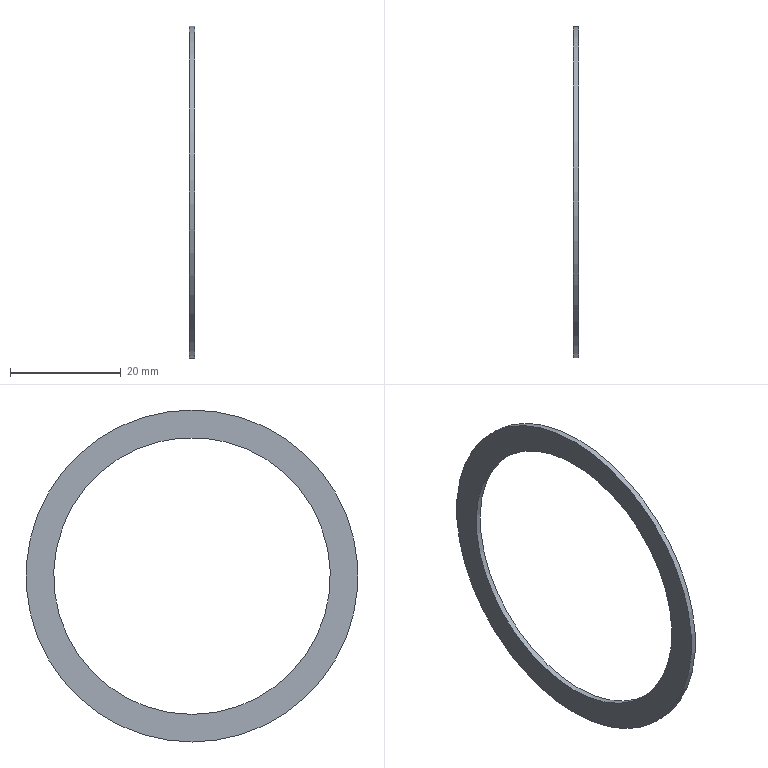Component | NX | GASKET | 1 solid | 4 faces | box 1 x 60 x 60 mm | volume 864 mm3 | cylinder 2 | plane 2 | commonest cylinder face diameters 60 x1 50 x1
STEP:
#1=CARTESIAN_POINT('',(0.,0.,0.));
#2=DIRECTION('',(0.,0.,1.));
#3=DIRECTION('',(1.,0.,0.));
#4=AXIS2_PLACEMENT_3D('',#1,#2,#3);
#5=CARTESIAN_POINT('',(144.,0.,-30.));
#6=VERTEX_POINT('',#5);
#7=CARTESIAN_POINT('',(144.,0.,0.));
#8=DIRECTION('',(1.,0.,0.));
#9=DIRECTION('',(0.,0.,-1.));
#10=AXIS2_PLACEMENT_3D('',#7,#8,#9);
#11=CIRCLE('',#10,30.);
#12=CARTESIAN_POINT('',(144.,0.,0.));
#13=DIRECTION('',(-1.,0.,0.));
#14=DIRECTION('',(0.,0.,1.));
#15=AXIS2_PLACEMENT_3D('',#12,#13,#14);
#16=CYLINDRICAL_SURFACE('',#15,30.);
#17=CARTESIAN_POINT('',(9.425,0.));
#18=DIRECTION('',(-1.,0.));
#19=VECTOR('',#18,1.);
#20=LINE('',#17,#19);
#21=(GEOMETRIC_REPRESENTATION_CONTEXT(2)PARAMETRIC_REPRESENTATION_CONTEXT()REPRESENTATION_CONTEXT('',''));
#22=DEFINITIONAL_REPRESENTATION('',(#20),#21);
#23=PCURVE('',#16,#22);
#24=CARTESIAN_POINT('',(144.,0.,0.));
#25=DIRECTION('',(1.,0.,0.));
#26=DIRECTION('',(0.,0.,-1.));
#27=AXIS2_PLACEMENT_3D('',#24,#25,#26);
#28=PLANE('',#27);
#29=CARTESIAN_POINT('',(0.,0.));
#30=DIRECTION('',(1.,0.));
#31=AXIS2_PLACEMENT_2D('',#29,#30);
#32=CIRCLE('',#31,30.);
#33=(GEOMETRIC_REPRESENTATION_CONTEXT(2)PARAMETRIC_REPRESENTATION_CONTEXT()REPRESENTATION_CONTEXT('',''));
#34=DEFINITIONAL_REPRESENTATION('',(#32),#33);
#35=PCURVE('',#28,#34);
#36=SURFACE_CURVE('',#11,(#23,#35),.PCURVE_S1.);
#37=EDGE_CURVE('',#6,#6,#36,.T.);
#38=ORIENTED_EDGE('',*,*,#37,.F.);
#39=CARTESIAN_POINT('',(143.,0.,-30.));
#40=VERTEX_POINT('',#39);
#41=CARTESIAN_POINT('',(144.,0.,-30.));
#42=CARTESIAN_POINT('',(143.,0.,-30.));
#43=B_SPLINE_CURVE_WITH_KNOTS('',1,(#41,#42),.UNSPECIFIED.,.F.,.F.,(2,2),(0.,1.),.PIECEWISE_BEZIER_KNOTS.);
#44=CARTESIAN_POINT('',(9.425,0.));
#45=DIRECTION('',(0.,1.));
#46=VECTOR('',#45,1.);
#47=LINE('',#44,#46);
#48=(GEOMETRIC_REPRESENTATION_CONTEXT(2)PARAMETRIC_REPRESENTATION_CONTEXT()REPRESENTATION_CONTEXT('',''));
#49=DEFINITIONAL_REPRESENTATION('',(#47),#48);
#50=PCURVE('',#16,#49);
#51=CARTESIAN_POINT('',(3.142,0.));
#52=DIRECTION('',(0.,1.));
#53=VECTOR('',#52,1.);
#54=LINE('',#51,#53);
#55=(GEOMETRIC_REPRESENTATION_CONTEXT(2)PARAMETRIC_REPRESENTATION_CONTEXT()REPRESENTATION_CONTEXT('',''));
#56=DEFINITIONAL_REPRESENTATION('',(#54),#55);
#57=PCURVE('',#16,#56);
#58=SEAM_CURVE('',#43,(#50,#57),.PCURVE_S1.);
#59=EDGE_CURVE('',#6,#40,#58,.T.);
#60=ORIENTED_EDGE('',*,*,#59,.T.);
#61=CARTESIAN_POINT('',(143.,0.,0.));
#62=DIRECTION('',(1.,0.,0.));
#63=DIRECTION('',(0.,0.,-1.));
#64=AXIS2_PLACEMENT_3D('',#61,#62,#63);
#65=CIRCLE('',#64,30.);
#66=CARTESIAN_POINT('',(9.425,1.));
#67=DIRECTION('',(-1.,0.));
#68=VECTOR('',#67,1.);
#69=LINE('',#66,#68);
#70=(GEOMETRIC_REPRESENTATION_CONTEXT(2)PARAMETRIC_REPRESENTATION_CONTEXT()REPRESENTATION_CONTEXT('',''));
#71=DEFINITIONAL_REPRESENTATION('',(#69),#70);
#72=PCURVE('',#16,#71);
#73=CARTESIAN_POINT('',(143.,0.,0.));
#74=DIRECTION('',(1.,0.,0.));
#75=DIRECTION('',(0.,0.,-1.));
#76=AXIS2_PLACEMENT_3D('',#73,#74,#75);
#77=PLANE('',#76);
#78=CARTESIAN_POINT('',(0.,0.));
#79=DIRECTION('',(1.,0.));
#80=AXIS2_PLACEMENT_2D('',#78,#79);
#81=CIRCLE('',#80,30.);
#82=(GEOMETRIC_REPRESENTATION_CONTEXT(2)PARAMETRIC_REPRESENTATION_CONTEXT()REPRESENTATION_CONTEXT('',''));
#83=DEFINITIONAL_REPRESENTATION('',(#81),#82);
#84=PCURVE('',#77,#83);
#85=SURFACE_CURVE('',#65,(#72,#84),.PCURVE_S1.);
#86=EDGE_CURVE('',#40,#40,#85,.T.);
#87=ORIENTED_EDGE('',*,*,#86,.T.);
#88=ORIENTED_EDGE('',*,*,#59,.F.);
#89=EDGE_LOOP('',(#38,#60,#87,#88));
#90=FACE_BOUND('',#89,.T.);
#91=ADVANCED_FACE('',(#90),#16,.T.);
#92=CARTESIAN_POINT('',(144.,0.,-25.));
#93=VERTEX_POINT('',#92);
#94=CARTESIAN_POINT('',(144.,0.,0.));
#95=DIRECTION('',(1.,0.,0.));
#96=DIRECTION('',(0.,0.,-1.));
#97=AXIS2_PLACEMENT_3D('',#94,#95,#96);
#98=CIRCLE('',#97,25.);
#99=CARTESIAN_POINT('',(144.,0.,0.));
#100=DIRECTION('',(-1.,0.,0.));
#101=DIRECTION('',(0.,0.,1.));
#102=AXIS2_PLACEMENT_3D('',#99,#100,#101);
#103=CYLINDRICAL_SURFACE('',#102,25.);
#104=CARTESIAN_POINT('',(9.425,0.));
#105=DIRECTION('',(-1.,0.));
#106=VECTOR('',#105,1.);
#107=LINE('',#104,#106);
#108=(GEOMETRIC_REPRESENTATION_CONTEXT(2)PARAMETRIC_REPRESENTATION_CONTEXT()REPRESENTATION_CONTEXT('',''));
#109=DEFINITIONAL_REPRESENTATION('',(#107),#108);
#110=PCURVE('',#103,#109);
#111=CARTESIAN_POINT('',(0.,0.));
#112=DIRECTION('',(1.,0.));
#113=AXIS2_PLACEMENT_2D('',#111,#112);
#114=CIRCLE('',#113,25.);
#115=(GEOMETRIC_REPRESENTATION_CONTEXT(2)PARAMETRIC_REPRESENTATION_CONTEXT()REPRESENTATION_CONTEXT('',''));
#116=DEFINITIONAL_REPRESENTATION('',(#114),#115);
#117=PCURVE('',#28,#116);
#118=SURFACE_CURVE('',#98,(#110,#117),.PCURVE_S1.);
#119=EDGE_CURVE('',#93,#93,#118,.T.);
#120=ORIENTED_EDGE('',*,*,#119,.F.);
#121=CARTESIAN_POINT('',(143.,0.,-25.));
#122=VERTEX_POINT('',#121);
#123=CARTESIAN_POINT('',(144.,0.,-25.));
#124=CARTESIAN_POINT('',(143.,0.,-25.));
#125=B_SPLINE_CURVE_WITH_KNOTS('',1,(#123,#124),.UNSPECIFIED.,.F.,.F.,(2,2),(0.,1.),.PIECEWISE_BEZIER_KNOTS.);
#126=CARTESIAN_POINT('',(9.425,0.));
#127=DIRECTION('',(0.,1.));
#128=VECTOR('',#127,1.);
#129=LINE('',#126,#128);
#130=(GEOMETRIC_REPRESENTATION_CONTEXT(2)PARAMETRIC_REPRESENTATION_CONTEXT()REPRESENTATION_CONTEXT('',''));
#131=DEFINITIONAL_REPRESENTATION('',(#129),#130);
#132=PCURVE('',#103,#131);
#133=CARTESIAN_POINT('',(3.142,0.));
#134=DIRECTION('',(0.,1.));
#135=VECTOR('',#134,1.);
#136=LINE('',#133,#135);
#137=(GEOMETRIC_REPRESENTATION_CONTEXT(2)PARAMETRIC_REPRESENTATION_CONTEXT()REPRESENTATION_CONTEXT('',''));
#138=DEFINITIONAL_REPRESENTATION('',(#136),#137);
#139=PCURVE('',#103,#138);
#140=SEAM_CURVE('',#125,(#132,#139),.PCURVE_S1.);
#141=EDGE_CURVE('',#93,#122,#140,.T.);
#142=ORIENTED_EDGE('',*,*,#141,.T.);
#143=CARTESIAN_POINT('',(143.,0.,0.));
#144=DIRECTION('',(1.,0.,0.));
#145=DIRECTION('',(0.,0.,-1.));
#146=AXIS2_PLACEMENT_3D('',#143,#144,#145);
#147=CIRCLE('',#146,25.);
#148=CARTESIAN_POINT('',(9.425,1.));
#149=DIRECTION('',(-1.,0.));
#150=VECTOR('',#149,1.);
#151=LINE('',#148,#150);
#152=(GEOMETRIC_REPRESENTATION_CONTEXT(2)PARAMETRIC_REPRESENTATION_CONTEXT()REPRESENTATION_CONTEXT('',''));
#153=DEFINITIONAL_REPRESENTATION('',(#151),#152);
#154=PCURVE('',#103,#153);
#155=CARTESIAN_POINT('',(0.,0.));
#156=DIRECTION('',(1.,0.));
#157=AXIS2_PLACEMENT_2D('',#155,#156);
#158=CIRCLE('',#157,25.);
#159=(GEOMETRIC_REPRESENTATION_CONTEXT(2)PARAMETRIC_REPRESENTATION_CONTEXT()REPRESENTATION_CONTEXT('',''));
#160=DEFINITIONAL_REPRESENTATION('',(#158),#159);
#161=PCURVE('',#77,#160);
#162=SURFACE_CURVE('',#147,(#154,#161),.PCURVE_S1.);
#163=EDGE_CURVE('',#122,#122,#162,.T.);
#164=ORIENTED_EDGE('',*,*,#163,.T.);
#165=ORIENTED_EDGE('',*,*,#141,.F.);
#166=EDGE_LOOP('',(#120,#142,#164,#165));
#167=FACE_BOUND('',#166,.F.);
#168=ADVANCED_FACE('',(#167),#103,.F.);
#169=ORIENTED_EDGE('',*,*,#37,.T.);
#170=EDGE_LOOP('',(#169));
#171=FACE_BOUND('',#170,.T.);
#172=ORIENTED_EDGE('',*,*,#119,.F.);
#173=EDGE_LOOP('',(#172));
#174=FACE_BOUND('',#173,.T.);
#175=ADVANCED_FACE('',(#171,#174),#28,.T.);
#176=ORIENTED_EDGE('',*,*,#86,.F.);
#177=EDGE_LOOP('',(#176));
#178=FACE_BOUND('',#177,.T.);
#179=ORIENTED_EDGE('',*,*,#163,.T.);
#180=EDGE_LOOP('',(#179));
#181=FACE_BOUND('',#180,.T.);
#182=ADVANCED_FACE('',(#178,#181),#77,.F.);
#183=CLOSED_SHELL('',(#91,#168,#175,#182));
#184=MANIFOLD_SOLID_BREP('',#183);
#185=(LENGTH_UNIT()NAMED_UNIT(*)SI_UNIT(.MILLI.,.METRE.));
#186=UNCERTAINTY_MEASURE_WITH_UNIT(LENGTH_MEASURE(0.00001),#185,'','');
#187=(NAMED_UNIT(*)PLANE_ANGLE_UNIT()SI_UNIT($,.RADIAN.));
#188=(NAMED_UNIT(*)SI_UNIT($,.STERADIAN.)SOLID_ANGLE_UNIT());
#189=(GEOMETRIC_REPRESENTATION_CONTEXT(3)GLOBAL_UNCERTAINTY_ASSIGNED_CONTEXT((#186))GLOBAL_UNIT_ASSIGNED_CONTEXT((#185,#187,#188))REPRESENTATION_CONTEXT('',''));
#190=ADVANCED_BREP_SHAPE_REPRESENTATION('',(#4,#184),#189);